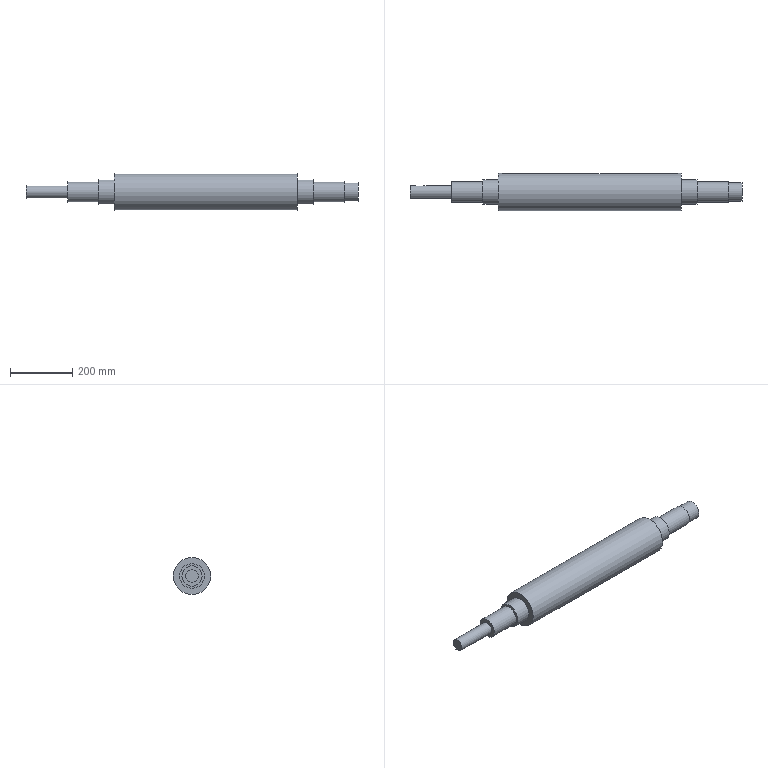Component | NX | MAIN_SHAFT | 1 solid | 25 faces | volume 7908147 mm3 | plane 14 | cylinder 11 | commonest cylinder face diameters 65 x2 80 x2 20 x2 15 x2 60 x1 120 x1 40 x1